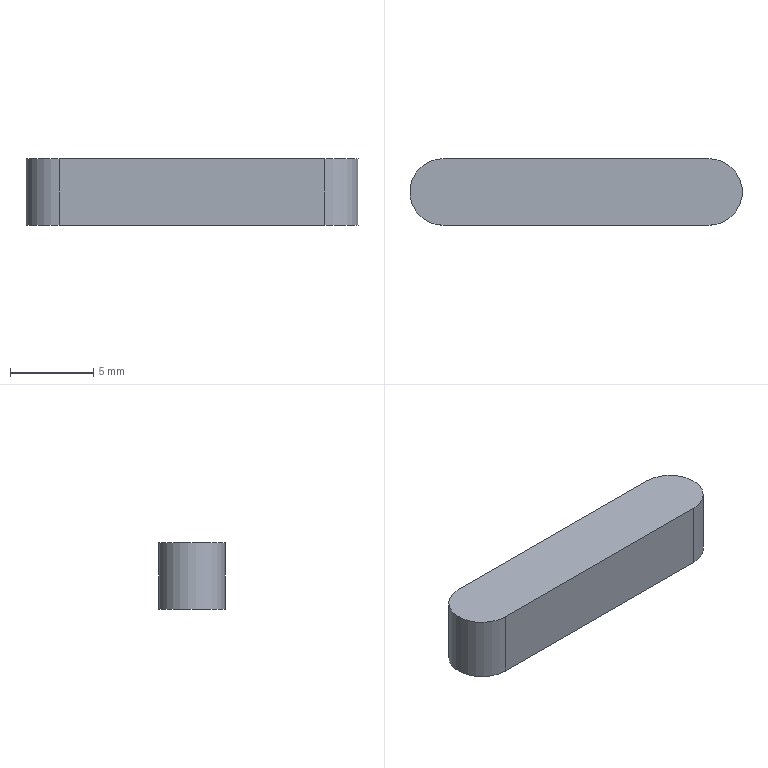Component | NX | FLAT_KEY | 1 solid | 6 faces | box 20 x 4 x 4 mm | volume 306 mm3 | plane 4 | cylinder 2 | commonest cylinder face diameters 4 x2
STEP:
#1=CARTESIAN_POINT('',(0.,0.,0.));
#2=DIRECTION('',(0.,0.,1.));
#3=DIRECTION('',(1.,0.,0.));
#4=AXIS2_PLACEMENT_3D('',#1,#2,#3);
#5=CARTESIAN_POINT('',(249.5,-2.,153.5));
#6=VERTEX_POINT('',#5);
#7=CARTESIAN_POINT('',(249.5,2.,153.5));
#8=VERTEX_POINT('',#7);
#9=CARTESIAN_POINT('',(249.5,-0.,153.5));
#10=DIRECTION('',(0.,0.,1.));
#11=DIRECTION('',(1.,0.,0.));
#12=AXIS2_PLACEMENT_3D('',#9,#10,#11);
#13=CIRCLE('',#12,2.);
#14=CARTESIAN_POINT('',(241.5,-0.,153.5));
#15=DIRECTION('',(0.,0.,1.));
#16=DIRECTION('',(1.,0.,0.));
#17=AXIS2_PLACEMENT_3D('',#14,#15,#16);
#18=PLANE('',#17);
#19=CARTESIAN_POINT('',(8.,0.));
#20=DIRECTION('',(1.,0.));
#21=AXIS2_PLACEMENT_2D('',#19,#20);
#22=CIRCLE('',#21,2.);
#23=(GEOMETRIC_REPRESENTATION_CONTEXT(2)PARAMETRIC_REPRESENTATION_CONTEXT()REPRESENTATION_CONTEXT('',''));
#24=DEFINITIONAL_REPRESENTATION('',(#22),#23);
#25=PCURVE('',#18,#24);
#26=CARTESIAN_POINT('',(249.5,-0.,149.5));
#27=DIRECTION('',(0.,0.,1.));
#28=DIRECTION('',(1.,0.,0.));
#29=AXIS2_PLACEMENT_3D('',#26,#27,#28);
#30=CYLINDRICAL_SURFACE('',#29,2.);
#31=CARTESIAN_POINT('',(0.,4.));
#32=DIRECTION('',(1.,0.));
#33=VECTOR('',#32,1.);
#34=LINE('',#31,#33);
#35=(GEOMETRIC_REPRESENTATION_CONTEXT(2)PARAMETRIC_REPRESENTATION_CONTEXT()REPRESENTATION_CONTEXT('',''));
#36=DEFINITIONAL_REPRESENTATION('',(#34),#35);
#37=PCURVE('',#30,#36);
#38=SURFACE_CURVE('',#13,(#25,#37),.PCURVE_S1.);
#39=EDGE_CURVE('',#6,#8,#38,.T.);
#40=ORIENTED_EDGE('',*,*,#39,.T.);
#41=CARTESIAN_POINT('',(233.5,2.,153.5));
#42=VERTEX_POINT('',#41);
#43=CARTESIAN_POINT('',(241.5,2.,153.5));
#44=DIRECTION('',(1.,0.,0.));
#45=VECTOR('',#44,1.);
#46=LINE('',#43,#45);
#47=CARTESIAN_POINT('',(0.,2.));
#48=DIRECTION('',(1.,0.));
#49=VECTOR('',#48,1.);
#50=LINE('',#47,#49);
#51=(GEOMETRIC_REPRESENTATION_CONTEXT(2)PARAMETRIC_REPRESENTATION_CONTEXT()REPRESENTATION_CONTEXT('',''));
#52=DEFINITIONAL_REPRESENTATION('',(#50),#51);
#53=PCURVE('',#18,#52);
#54=CARTESIAN_POINT('',(241.5,2.,149.5));
#55=DIRECTION('',(0.,1.,0.));
#56=DIRECTION('',(0.,0.,1.));
#57=AXIS2_PLACEMENT_3D('',#54,#55,#56);
#58=PLANE('',#57);
#59=CARTESIAN_POINT('',(4.,0.));
#60=DIRECTION('',(0.,1.));
#61=VECTOR('',#60,1.);
#62=LINE('',#59,#61);
#63=(GEOMETRIC_REPRESENTATION_CONTEXT(2)PARAMETRIC_REPRESENTATION_CONTEXT()REPRESENTATION_CONTEXT('',''));
#64=DEFINITIONAL_REPRESENTATION('',(#62),#63);
#65=PCURVE('',#58,#64);
#66=SURFACE_CURVE('',#46,(#53,#65),.PCURVE_S1.);
#67=EDGE_CURVE('',#42,#8,#66,.T.);
#68=ORIENTED_EDGE('',*,*,#67,.F.);
#69=CARTESIAN_POINT('',(233.5,-2.,153.5));
#70=VERTEX_POINT('',#69);
#71=CARTESIAN_POINT('',(233.5,-0.,153.5));
#72=DIRECTION('',(0.,0.,1.));
#73=DIRECTION('',(1.,0.,0.));
#74=AXIS2_PLACEMENT_3D('',#71,#72,#73);
#75=CIRCLE('',#74,2.);
#76=CARTESIAN_POINT('',(-8.,0.));
#77=DIRECTION('',(1.,0.));
#78=AXIS2_PLACEMENT_2D('',#76,#77);
#79=CIRCLE('',#78,2.);
#80=(GEOMETRIC_REPRESENTATION_CONTEXT(2)PARAMETRIC_REPRESENTATION_CONTEXT()REPRESENTATION_CONTEXT('',''));
#81=DEFINITIONAL_REPRESENTATION('',(#79),#80);
#82=PCURVE('',#18,#81);
#83=CARTESIAN_POINT('',(233.5,-0.,149.5));
#84=DIRECTION('',(0.,0.,1.));
#85=DIRECTION('',(1.,0.,0.));
#86=AXIS2_PLACEMENT_3D('',#83,#84,#85);
#87=CYLINDRICAL_SURFACE('',#86,2.);
#88=CARTESIAN_POINT('',(0.,4.));
#89=DIRECTION('',(1.,0.));
#90=VECTOR('',#89,1.);
#91=LINE('',#88,#90);
#92=(GEOMETRIC_REPRESENTATION_CONTEXT(2)PARAMETRIC_REPRESENTATION_CONTEXT()REPRESENTATION_CONTEXT('',''));
#93=DEFINITIONAL_REPRESENTATION('',(#91),#92);
#94=PCURVE('',#87,#93);
#95=SURFACE_CURVE('',#75,(#82,#94),.PCURVE_S1.);
#96=EDGE_CURVE('',#42,#70,#95,.T.);
#97=ORIENTED_EDGE('',*,*,#96,.T.);
#98=CARTESIAN_POINT('',(241.5,-2.,153.5));
#99=DIRECTION('',(-1.,0.,0.));
#100=VECTOR('',#99,1.);
#101=LINE('',#98,#100);
#102=CARTESIAN_POINT('',(0.,-2.));
#103=DIRECTION('',(-1.,0.));
#104=VECTOR('',#103,1.);
#105=LINE('',#102,#104);
#106=(GEOMETRIC_REPRESENTATION_CONTEXT(2)PARAMETRIC_REPRESENTATION_CONTEXT()REPRESENTATION_CONTEXT('',''));
#107=DEFINITIONAL_REPRESENTATION('',(#105),#106);
#108=PCURVE('',#18,#107);
#109=CARTESIAN_POINT('',(241.5,-2.,149.5));
#110=DIRECTION('',(0.,-1.,0.));
#111=DIRECTION('',(0.,0.,-1.));
#112=AXIS2_PLACEMENT_3D('',#109,#110,#111);
#113=PLANE('',#112);
#114=CARTESIAN_POINT('',(-4.,0.));
#115=DIRECTION('',(0.,-1.));
#116=VECTOR('',#115,1.);
#117=LINE('',#114,#116);
#118=(GEOMETRIC_REPRESENTATION_CONTEXT(2)PARAMETRIC_REPRESENTATION_CONTEXT()REPRESENTATION_CONTEXT('',''));
#119=DEFINITIONAL_REPRESENTATION('',(#117),#118);
#120=PCURVE('',#113,#119);
#121=SURFACE_CURVE('',#101,(#108,#120),.PCURVE_S1.);
#122=EDGE_CURVE('',#6,#70,#121,.T.);
#123=ORIENTED_EDGE('',*,*,#122,.F.);
#124=EDGE_LOOP('',(#40,#68,#97,#123));
#125=FACE_BOUND('',#124,.T.);
#126=ADVANCED_FACE('',(#125),#18,.T.);
#127=CARTESIAN_POINT('',(233.5,-2.,149.5));
#128=VERTEX_POINT('',#127);
#129=CARTESIAN_POINT('',(249.5,-2.,149.5));
#130=VERTEX_POINT('',#129);
#131=CARTESIAN_POINT('',(241.5,-2.,149.5));
#132=DIRECTION('',(1.,0.,0.));
#133=VECTOR('',#132,1.);
#134=LINE('',#131,#133);
#135=CARTESIAN_POINT('',(0.,0.));
#136=DIRECTION('',(0.,1.));
#137=VECTOR('',#136,1.);
#138=LINE('',#135,#137);
#139=(GEOMETRIC_REPRESENTATION_CONTEXT(2)PARAMETRIC_REPRESENTATION_CONTEXT()REPRESENTATION_CONTEXT('',''));
#140=DEFINITIONAL_REPRESENTATION('',(#138),#139);
#141=PCURVE('',#113,#140);
#142=CARTESIAN_POINT('',(241.5,-0.,149.5));
#143=DIRECTION('',(0.,0.,-1.));
#144=DIRECTION('',(-1.,0.,0.));
#145=AXIS2_PLACEMENT_3D('',#142,#143,#144);
#146=PLANE('',#145);
#147=CARTESIAN_POINT('',(0.,-2.));
#148=DIRECTION('',(-1.,0.));
#149=VECTOR('',#148,1.);
#150=LINE('',#147,#149);
#151=(GEOMETRIC_REPRESENTATION_CONTEXT(2)PARAMETRIC_REPRESENTATION_CONTEXT()REPRESENTATION_CONTEXT('',''));
#152=DEFINITIONAL_REPRESENTATION('',(#150),#151);
#153=PCURVE('',#146,#152);
#154=SURFACE_CURVE('',#134,(#141,#153),.PCURVE_S1.);
#155=EDGE_CURVE('',#128,#130,#154,.T.);
#156=ORIENTED_EDGE('',*,*,#155,.T.);
#157=CARTESIAN_POINT('',(249.5,-2.,149.5));
#158=DIRECTION('',(0.,0.,1.));
#159=VECTOR('',#158,1.);
#160=LINE('',#157,#159);
#161=CARTESIAN_POINT('',(0.,8.));
#162=DIRECTION('',(-1.,0.));
#163=VECTOR('',#162,1.);
#164=LINE('',#161,#163);
#165=(GEOMETRIC_REPRESENTATION_CONTEXT(2)PARAMETRIC_REPRESENTATION_CONTEXT()REPRESENTATION_CONTEXT('',''));
#166=DEFINITIONAL_REPRESENTATION('',(#164),#165);
#167=PCURVE('',#113,#166);
#168=CARTESIAN_POINT('',(4.712,0.));
#169=DIRECTION('',(0.,1.));
#170=VECTOR('',#169,1.);
#171=LINE('',#168,#170);
#172=(GEOMETRIC_REPRESENTATION_CONTEXT(2)PARAMETRIC_REPRESENTATION_CONTEXT()REPRESENTATION_CONTEXT('',''));
#173=DEFINITIONAL_REPRESENTATION('',(#171),#172);
#174=PCURVE('',#30,#173);
#175=SURFACE_CURVE('',#160,(#167,#174),.PCURVE_S1.);
#176=EDGE_CURVE('',#130,#6,#175,.T.);
#177=ORIENTED_EDGE('',*,*,#176,.T.);
#178=ORIENTED_EDGE('',*,*,#122,.T.);
#179=CARTESIAN_POINT('',(233.5,-2.,149.5));
#180=DIRECTION('',(0.,0.,-1.));
#181=VECTOR('',#180,1.);
#182=LINE('',#179,#181);
#183=CARTESIAN_POINT('',(0.,-8.));
#184=DIRECTION('',(1.,0.));
#185=VECTOR('',#184,1.);
#186=LINE('',#183,#185);
#187=(GEOMETRIC_REPRESENTATION_CONTEXT(2)PARAMETRIC_REPRESENTATION_CONTEXT()REPRESENTATION_CONTEXT('',''));
#188=DEFINITIONAL_REPRESENTATION('',(#186),#187);
#189=PCURVE('',#113,#188);
#190=CARTESIAN_POINT('',(4.712,0.));
#191=DIRECTION('',(0.,-1.));
#192=VECTOR('',#191,1.);
#193=LINE('',#190,#192);
#194=(GEOMETRIC_REPRESENTATION_CONTEXT(2)PARAMETRIC_REPRESENTATION_CONTEXT()REPRESENTATION_CONTEXT('',''));
#195=DEFINITIONAL_REPRESENTATION('',(#193),#194);
#196=PCURVE('',#87,#195);
#197=SURFACE_CURVE('',#182,(#189,#196),.PCURVE_S1.);
#198=EDGE_CURVE('',#70,#128,#197,.T.);
#199=ORIENTED_EDGE('',*,*,#198,.T.);
#200=EDGE_LOOP('',(#156,#177,#178,#199));
#201=FACE_BOUND('',#200,.T.);
#202=ADVANCED_FACE('',(#201),#113,.T.);
#203=ORIENTED_EDGE('',*,*,#67,.T.);
#204=CARTESIAN_POINT('',(249.5,2.,149.5));
#205=VERTEX_POINT('',#204);
#206=CARTESIAN_POINT('',(249.5,2.,149.5));
#207=DIRECTION('',(0.,0.,-1.));
#208=VECTOR('',#207,1.);
#209=LINE('',#206,#208);
#210=CARTESIAN_POINT('',(0.,8.));
#211=DIRECTION('',(-1.,0.));
#212=VECTOR('',#211,1.);
#213=LINE('',#210,#212);
#214=(GEOMETRIC_REPRESENTATION_CONTEXT(2)PARAMETRIC_REPRESENTATION_CONTEXT()REPRESENTATION_CONTEXT('',''));
#215=DEFINITIONAL_REPRESENTATION('',(#213),#214);
#216=PCURVE('',#58,#215);
#217=CARTESIAN_POINT('',(7.854,0.));
#218=DIRECTION('',(0.,-1.));
#219=VECTOR('',#218,1.);
#220=LINE('',#217,#219);
#221=(GEOMETRIC_REPRESENTATION_CONTEXT(2)PARAMETRIC_REPRESENTATION_CONTEXT()REPRESENTATION_CONTEXT('',''));
#222=DEFINITIONAL_REPRESENTATION('',(#220),#221);
#223=PCURVE('',#30,#222);
#224=SURFACE_CURVE('',#209,(#216,#223),.PCURVE_S1.);
#225=EDGE_CURVE('',#8,#205,#224,.T.);
#226=ORIENTED_EDGE('',*,*,#225,.T.);
#227=CARTESIAN_POINT('',(233.5,2.,149.5));
#228=VERTEX_POINT('',#227);
#229=CARTESIAN_POINT('',(241.5,2.,149.5));
#230=DIRECTION('',(-1.,0.,0.));
#231=VECTOR('',#230,1.);
#232=LINE('',#229,#231);
#233=CARTESIAN_POINT('',(0.,0.));
#234=DIRECTION('',(0.,-1.));
#235=VECTOR('',#234,1.);
#236=LINE('',#233,#235);
#237=(GEOMETRIC_REPRESENTATION_CONTEXT(2)PARAMETRIC_REPRESENTATION_CONTEXT()REPRESENTATION_CONTEXT('',''));
#238=DEFINITIONAL_REPRESENTATION('',(#236),#237);
#239=PCURVE('',#58,#238);
#240=CARTESIAN_POINT('',(0.,2.));
#241=DIRECTION('',(1.,0.));
#242=VECTOR('',#241,1.);
#243=LINE('',#240,#242);
#244=(GEOMETRIC_REPRESENTATION_CONTEXT(2)PARAMETRIC_REPRESENTATION_CONTEXT()REPRESENTATION_CONTEXT('',''));
#245=DEFINITIONAL_REPRESENTATION('',(#243),#244);
#246=PCURVE('',#146,#245);
#247=SURFACE_CURVE('',#232,(#239,#246),.PCURVE_S1.);
#248=EDGE_CURVE('',#205,#228,#247,.T.);
#249=ORIENTED_EDGE('',*,*,#248,.T.);
#250=CARTESIAN_POINT('',(233.5,2.,149.5));
#251=DIRECTION('',(0.,0.,1.));
#252=VECTOR('',#251,1.);
#253=LINE('',#250,#252);
#254=CARTESIAN_POINT('',(0.,-8.));
#255=DIRECTION('',(1.,0.));
#256=VECTOR('',#255,1.);
#257=LINE('',#254,#256);
#258=(GEOMETRIC_REPRESENTATION_CONTEXT(2)PARAMETRIC_REPRESENTATION_CONTEXT()REPRESENTATION_CONTEXT('',''));
#259=DEFINITIONAL_REPRESENTATION('',(#257),#258);
#260=PCURVE('',#58,#259);
#261=CARTESIAN_POINT('',(1.571,0.));
#262=DIRECTION('',(0.,1.));
#263=VECTOR('',#262,1.);
#264=LINE('',#261,#263);
#265=(GEOMETRIC_REPRESENTATION_CONTEXT(2)PARAMETRIC_REPRESENTATION_CONTEXT()REPRESENTATION_CONTEXT('',''));
#266=DEFINITIONAL_REPRESENTATION('',(#264),#265);
#267=PCURVE('',#87,#266);
#268=SURFACE_CURVE('',#253,(#260,#267),.PCURVE_S1.);
#269=EDGE_CURVE('',#228,#42,#268,.T.);
#270=ORIENTED_EDGE('',*,*,#269,.T.);
#271=EDGE_LOOP('',(#203,#226,#249,#270));
#272=FACE_BOUND('',#271,.T.);
#273=ADVANCED_FACE('',(#272),#58,.T.);
#274=ORIENTED_EDGE('',*,*,#248,.F.);
#275=CARTESIAN_POINT('',(249.5,-0.,149.5));
#276=DIRECTION('',(0.,0.,-1.));
#277=DIRECTION('',(-1.,0.,0.));
#278=AXIS2_PLACEMENT_3D('',#275,#276,#277);
#279=CIRCLE('',#278,2.);
#280=CARTESIAN_POINT('',(-8.,0.));
#281=DIRECTION('',(1.,0.));
#282=AXIS2_PLACEMENT_2D('',#280,#281);
#283=CIRCLE('',#282,2.);
#284=(GEOMETRIC_REPRESENTATION_CONTEXT(2)PARAMETRIC_REPRESENTATION_CONTEXT()REPRESENTATION_CONTEXT('',''));
#285=DEFINITIONAL_REPRESENTATION('',(#283),#284);
#286=PCURVE('',#146,#285);
#287=CARTESIAN_POINT('',(9.425,0.));
#288=DIRECTION('',(-1.,0.));
#289=VECTOR('',#288,1.);
#290=LINE('',#287,#289);
#291=(GEOMETRIC_REPRESENTATION_CONTEXT(2)PARAMETRIC_REPRESENTATION_CONTEXT()REPRESENTATION_CONTEXT('',''));
#292=DEFINITIONAL_REPRESENTATION('',(#290),#291);
#293=PCURVE('',#30,#292);
#294=SURFACE_CURVE('',#279,(#286,#293),.PCURVE_S1.);
#295=EDGE_CURVE('',#205,#130,#294,.T.);
#296=ORIENTED_EDGE('',*,*,#295,.T.);
#297=ORIENTED_EDGE('',*,*,#155,.F.);
#298=CARTESIAN_POINT('',(233.5,-0.,149.5));
#299=DIRECTION('',(0.,0.,-1.));
#300=DIRECTION('',(-1.,0.,0.));
#301=AXIS2_PLACEMENT_3D('',#298,#299,#300);
#302=CIRCLE('',#301,2.);
#303=CARTESIAN_POINT('',(8.,0.));
#304=DIRECTION('',(1.,0.));
#305=AXIS2_PLACEMENT_2D('',#303,#304);
#306=CIRCLE('',#305,2.);
#307=(GEOMETRIC_REPRESENTATION_CONTEXT(2)PARAMETRIC_REPRESENTATION_CONTEXT()REPRESENTATION_CONTEXT('',''));
#308=DEFINITIONAL_REPRESENTATION('',(#306),#307);
#309=PCURVE('',#146,#308);
#310=CARTESIAN_POINT('',(9.425,0.));
#311=DIRECTION('',(-1.,0.));
#312=VECTOR('',#311,1.);
#313=LINE('',#310,#312);
#314=(GEOMETRIC_REPRESENTATION_CONTEXT(2)PARAMETRIC_REPRESENTATION_CONTEXT()REPRESENTATION_CONTEXT('',''));
#315=DEFINITIONAL_REPRESENTATION('',(#313),#314);
#316=PCURVE('',#87,#315);
#317=SURFACE_CURVE('',#302,(#309,#316),.PCURVE_S1.);
#318=EDGE_CURVE('',#128,#228,#317,.T.);
#319=ORIENTED_EDGE('',*,*,#318,.T.);
#320=EDGE_LOOP('',(#274,#296,#297,#319));
#321=FACE_BOUND('',#320,.T.);
#322=ADVANCED_FACE('',(#321),#146,.T.);
#323=ORIENTED_EDGE('',*,*,#176,.F.);
#324=ORIENTED_EDGE('',*,*,#295,.F.);
#325=ORIENTED_EDGE('',*,*,#225,.F.);
#326=ORIENTED_EDGE('',*,*,#39,.F.);
#327=EDGE_LOOP('',(#323,#324,#325,#326));
#328=FACE_BOUND('',#327,.T.);
#329=ADVANCED_FACE('',(#328),#30,.T.);
#330=ORIENTED_EDGE('',*,*,#96,.F.);
#331=ORIENTED_EDGE('',*,*,#269,.F.);
#332=ORIENTED_EDGE('',*,*,#318,.F.);
#333=ORIENTED_EDGE('',*,*,#198,.F.);
#334=EDGE_LOOP('',(#330,#331,#332,#333));
#335=FACE_BOUND('',#334,.T.);
#336=ADVANCED_FACE('',(#335),#87,.T.);
#337=CLOSED_SHELL('',(#126,#202,#273,#322,#329,#336));
#338=MANIFOLD_SOLID_BREP('',#337);
#339=(LENGTH_UNIT()NAMED_UNIT(*)SI_UNIT(.MILLI.,.METRE.));
#340=UNCERTAINTY_MEASURE_WITH_UNIT(LENGTH_MEASURE(0.0000001),#339,'','');
#341=(NAMED_UNIT(*)PLANE_ANGLE_UNIT()SI_UNIT($,.RADIAN.));
#342=(NAMED_UNIT(*)SI_UNIT($,.STERADIAN.)SOLID_ANGLE_UNIT());
#343=(GEOMETRIC_REPRESENTATION_CONTEXT(3)GLOBAL_UNCERTAINTY_ASSIGNED_CONTEXT((#340))GLOBAL_UNIT_ASSIGNED_CONTEXT((#339,#341,#342))REPRESENTATION_CONTEXT('',''));
#344=ADVANCED_BREP_SHAPE_REPRESENTATION('',(#4,#338),#343);